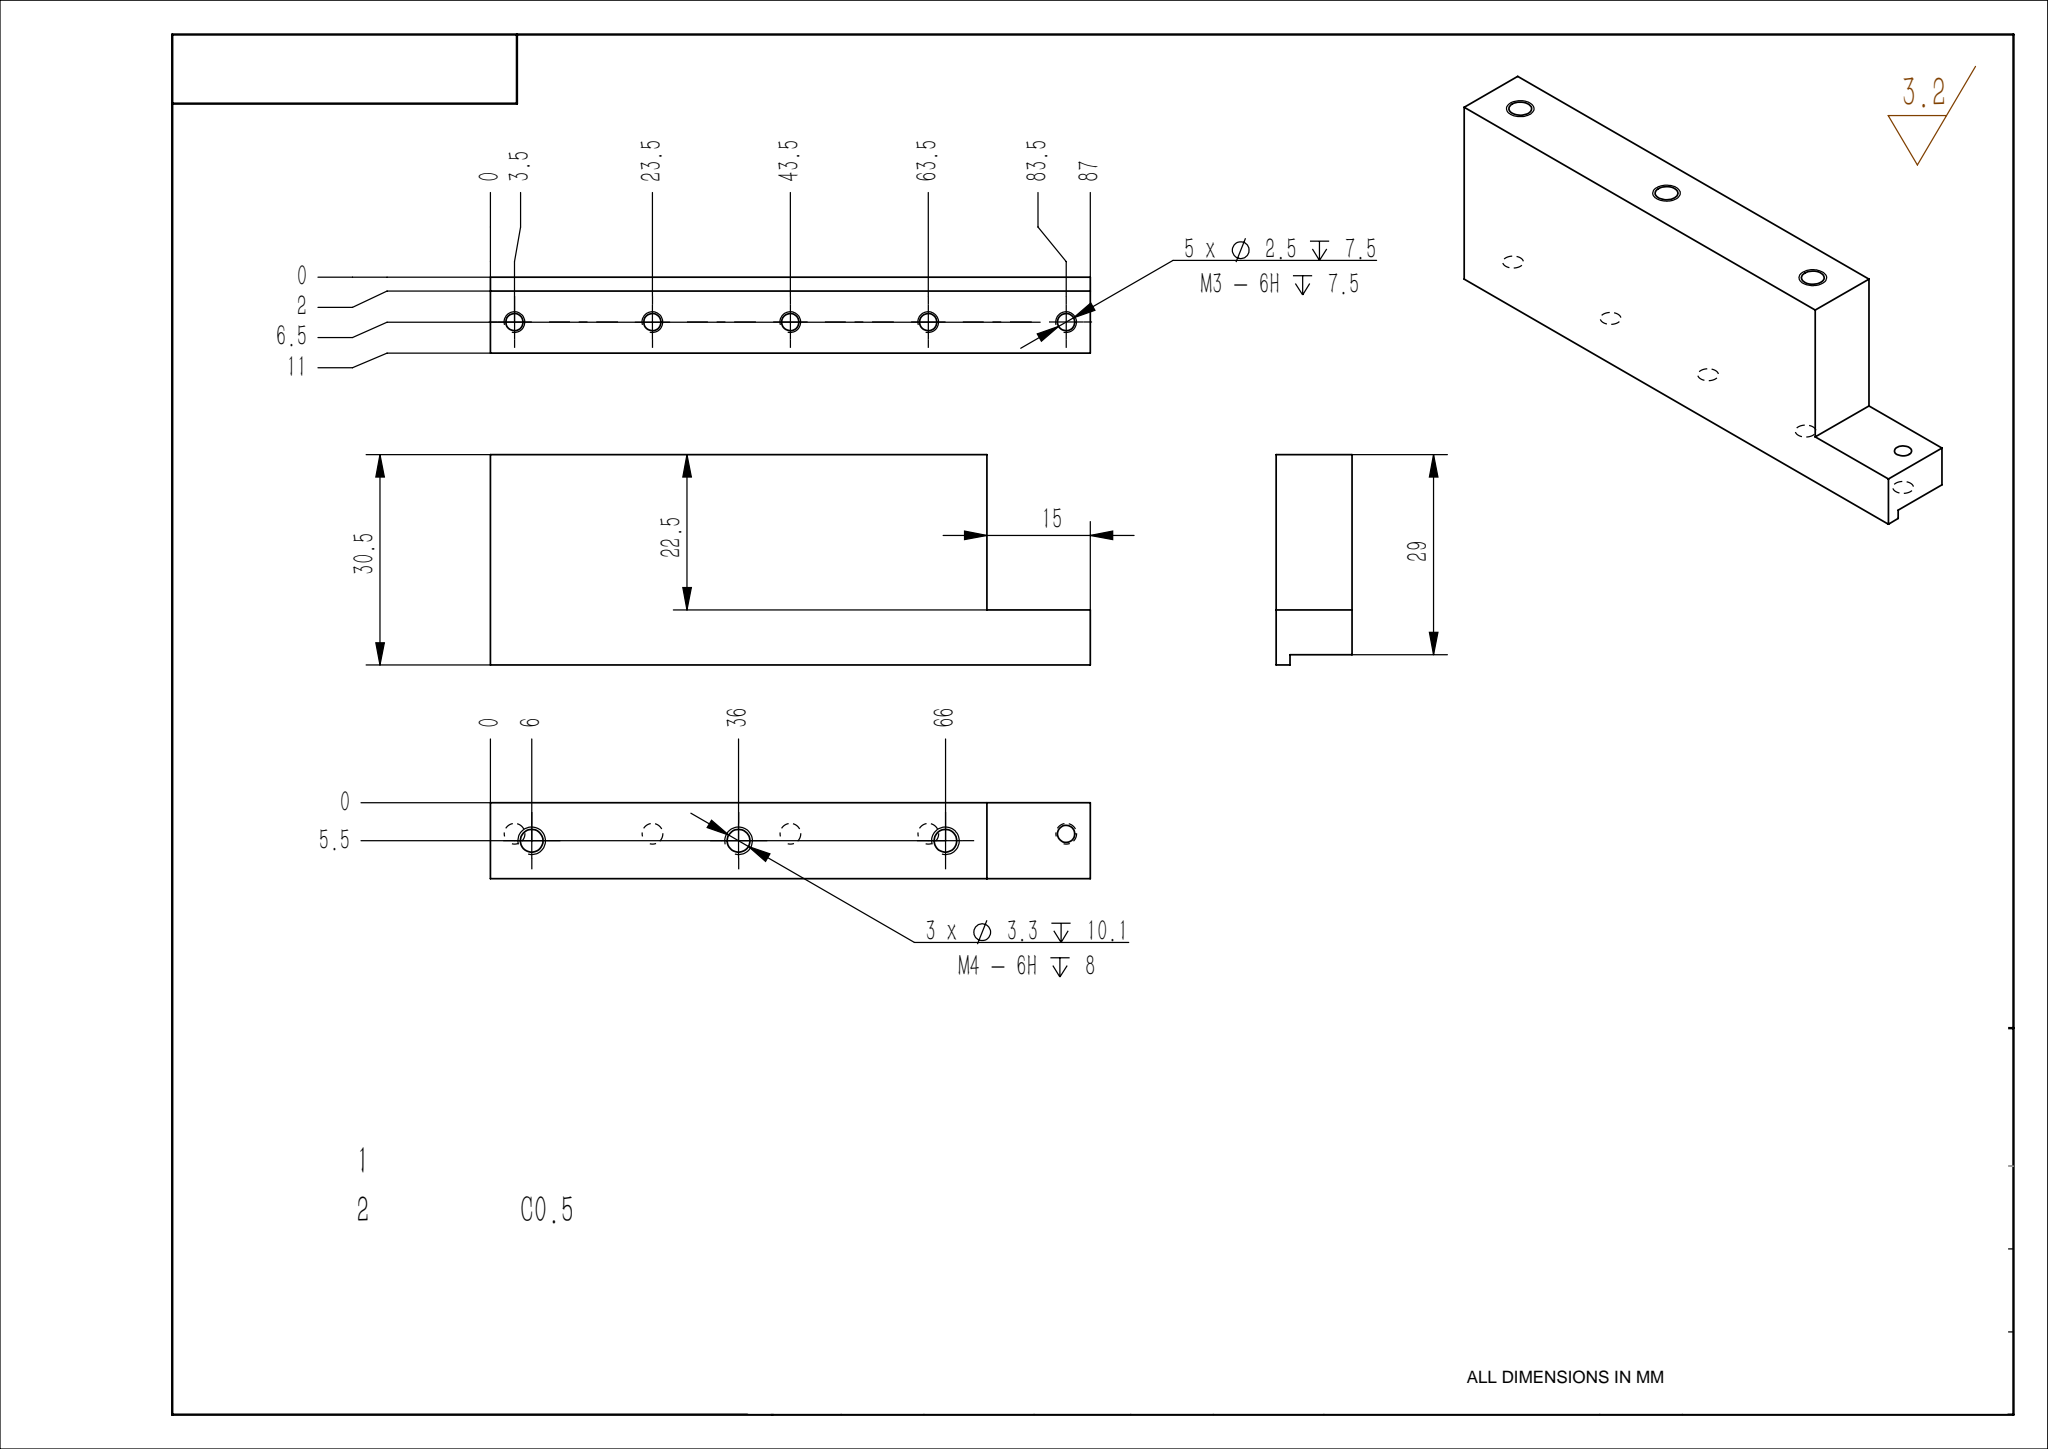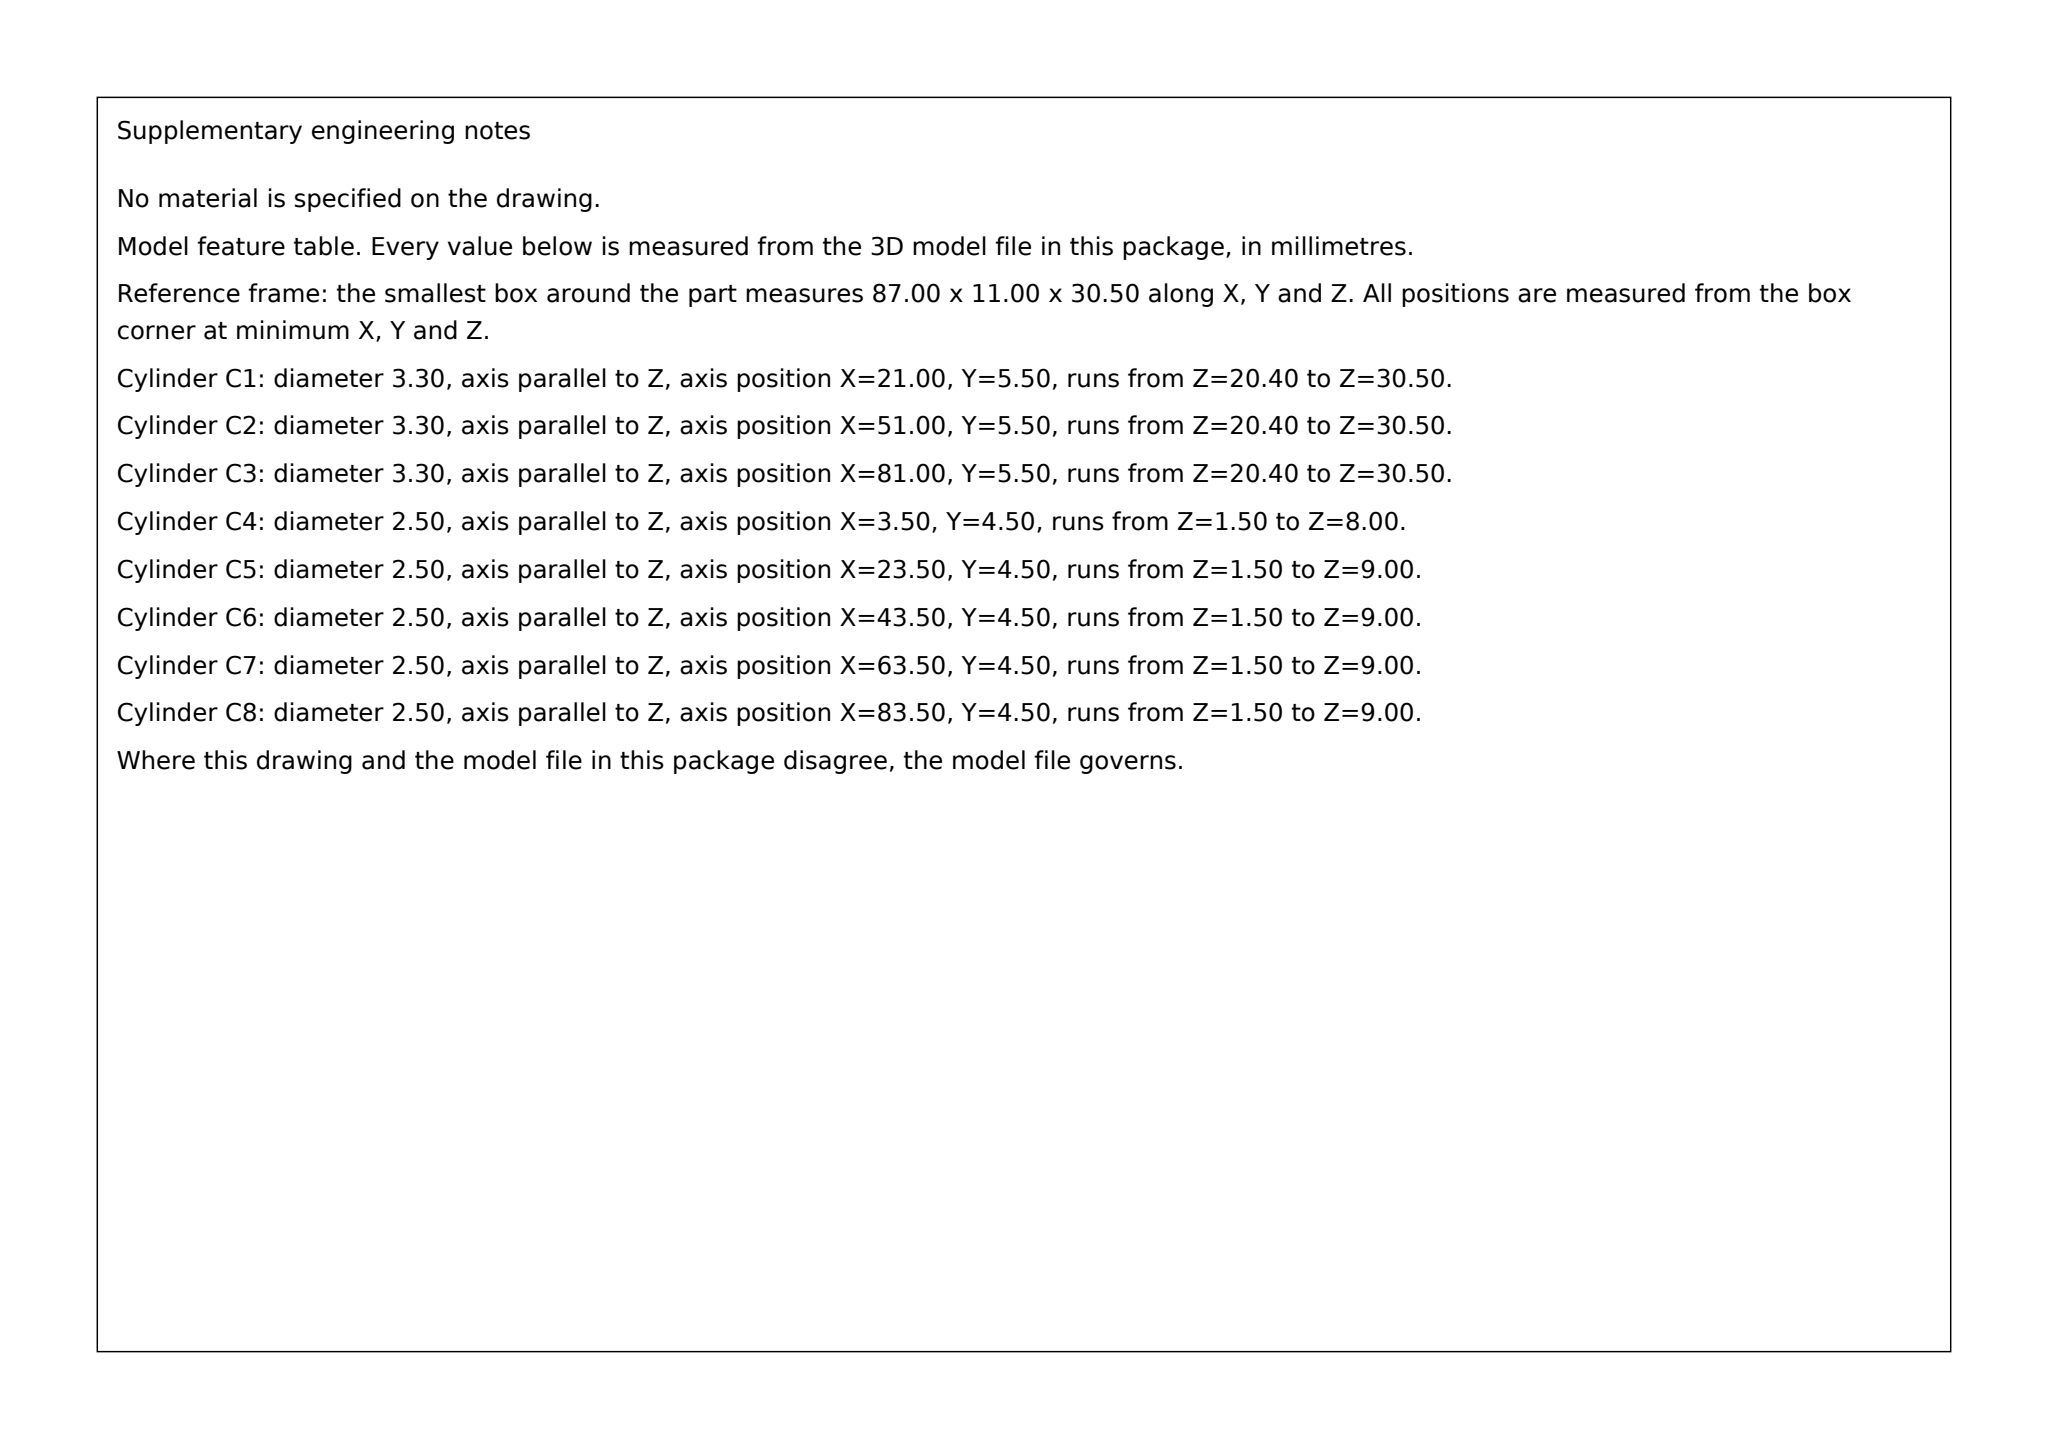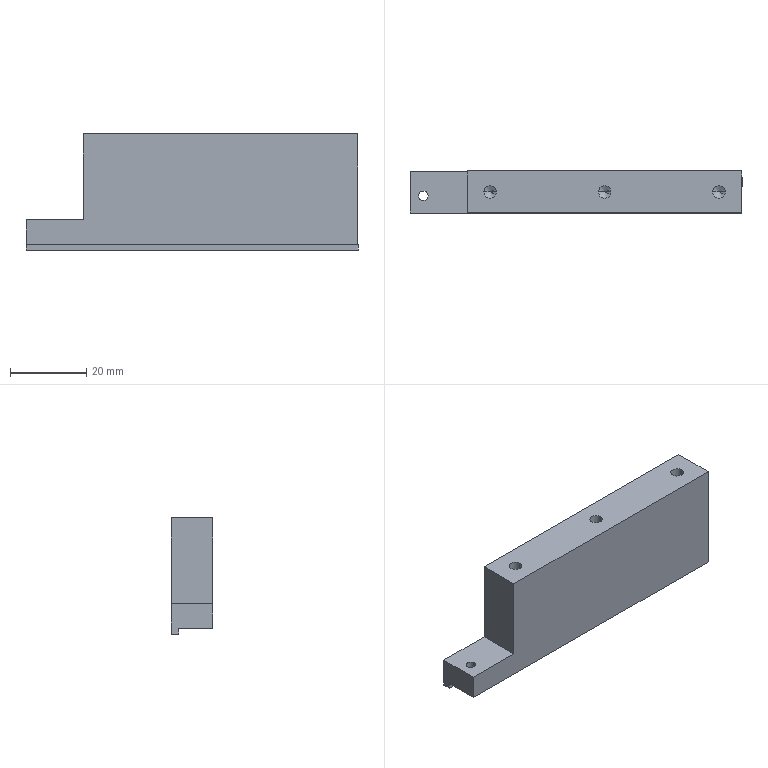Part | SolidWorks | mm | 1 solid | 40 faces | box 87 x 11 x 30.5 mm | volume 23850 mm3 | cylinder 16 | cone 14 | plane 10 | commonest cylinder face diameters 2.5 x10 3.3 x6
build123d program:
from build123d import *

# Parameters (mm, degrees)
SKETCH1_W             = 87
SKETCH1_H             = 30.5
BOSS_EXTRUDE1_DEPTH   = 11
SKETCH2_W             = 87
SKETCH2_H             = 9
CUT_EXTRUDE1_DEPTH    = 1.5
SKETCH3_W             = 23.872
SKETCH3_H             = 26.135
CUT_EXTRUDE2_DEPTH    = 48.39
LPATTERN1_COUNT       = 5
LPATTERN1_PITCH       = 20
M4_TAPPED_HOLE1_D     = 3.3
M4_TAPPED_HOLE1_DEPTH = 10.1
M4_TAPPED_HOLE1_TIP   = 0.9914


with BuildPart() as part:
    # Sketch1 → Boss-Extrude1 (new body)
    with BuildSketch(Plane(origin=(0, 0, 0), x_dir=(1, 0, 0), z_dir=(0, 1, 0))):
        Rectangle(SKETCH1_W, SKETCH1_H)
    extrude(amount=BOSS_EXTRUDE1_DEPTH)

    # Sketch2 → Cut-Extrude1 (cut)
    with BuildSketch(Plane(origin=(0, 0, -15.25), x_dir=(-1, 0, 0), z_dir=(0, 0, -1))):
        with Locations((0, 4.5)):
            Rectangle(SKETCH2_W, SKETCH2_H)
    extrude(amount=-CUT_EXTRUDE1_DEPTH, mode=Mode.SUBTRACT)

    # Sketch3 → Cut-Extrude2 (cut, through all)
    with BuildSketch(Plane(origin=(0, 11, 0), x_dir=(1, 0, 0), z_dir=(0, 1, 0))):
        with Locations((-40.436, -5.817)):
            Rectangle(SKETCH3_W, SKETCH3_H)
    extrude(amount=-CUT_EXTRUDE2_DEPTH, mode=Mode.SUBTRACT)

    # Sketch4 → M3 Tapped Hole1 (revolve, cut)
    with BuildSketch(Plane(origin=(40, 4.5, -13.75), x_dir=(0, 1, 0), z_dir=(1, 0, 0))):
        Polygon((0, 0), (0, 8.251), (1.25, 7.5), (1.25, 0), align=None)
    m3_tapped_hole1 = revolve(axis=Axis((40, 4.5, -20.1), (0, 0, 1)), mode=Mode.SUBTRACT)

    # LPattern1: M3 Tapped Hole1 ×5
    with Locations(*[(-i * LPATTERN1_PITCH, 0, 0) for i in range(1, LPATTERN1_COUNT)]):
        add(m3_tapped_hole1, mode=Mode.SUBTRACT)

    # M4 Tapped Hole1
    with Locations(Plane.XY.offset(15.25)):
        with Locations((-22.5, 5.5), (7.5, 5.5), (37.5, 5.5)):
            Hole(M4_TAPPED_HOLE1_D / 2, depth=M4_TAPPED_HOLE1_DEPTH)
            with Locations((0, 0, -(M4_TAPPED_HOLE1_DEPTH + M4_TAPPED_HOLE1_TIP / 2))):  # 118° drill point
                Cone(0, M4_TAPPED_HOLE1_D / 2, M4_TAPPED_HOLE1_TIP, mode=Mode.SUBTRACT)


solid = part.part